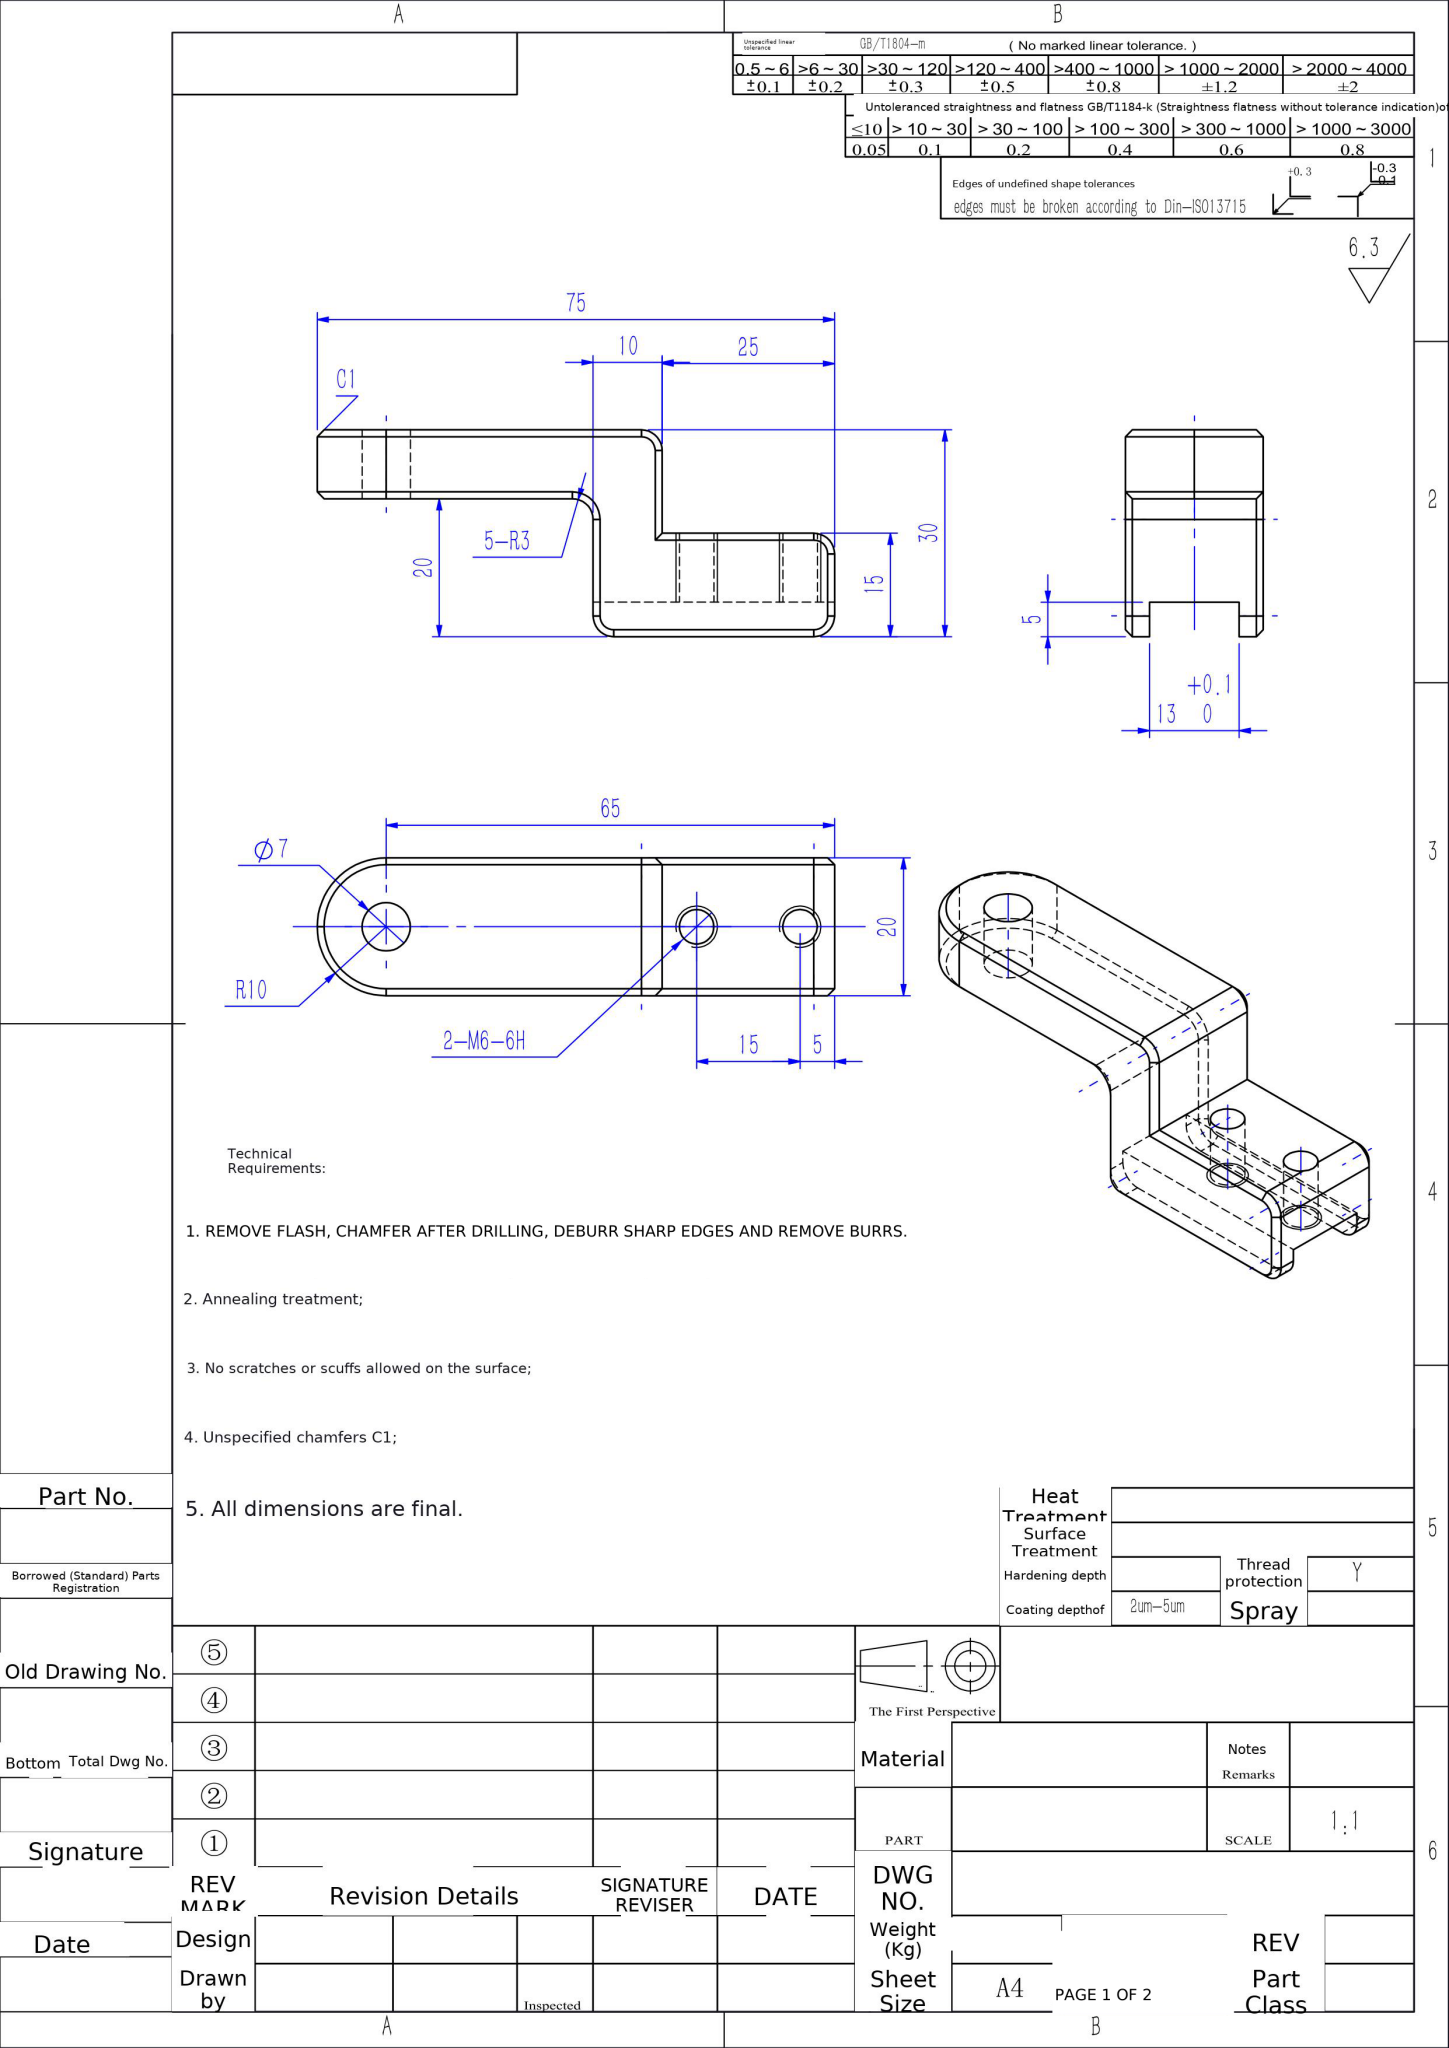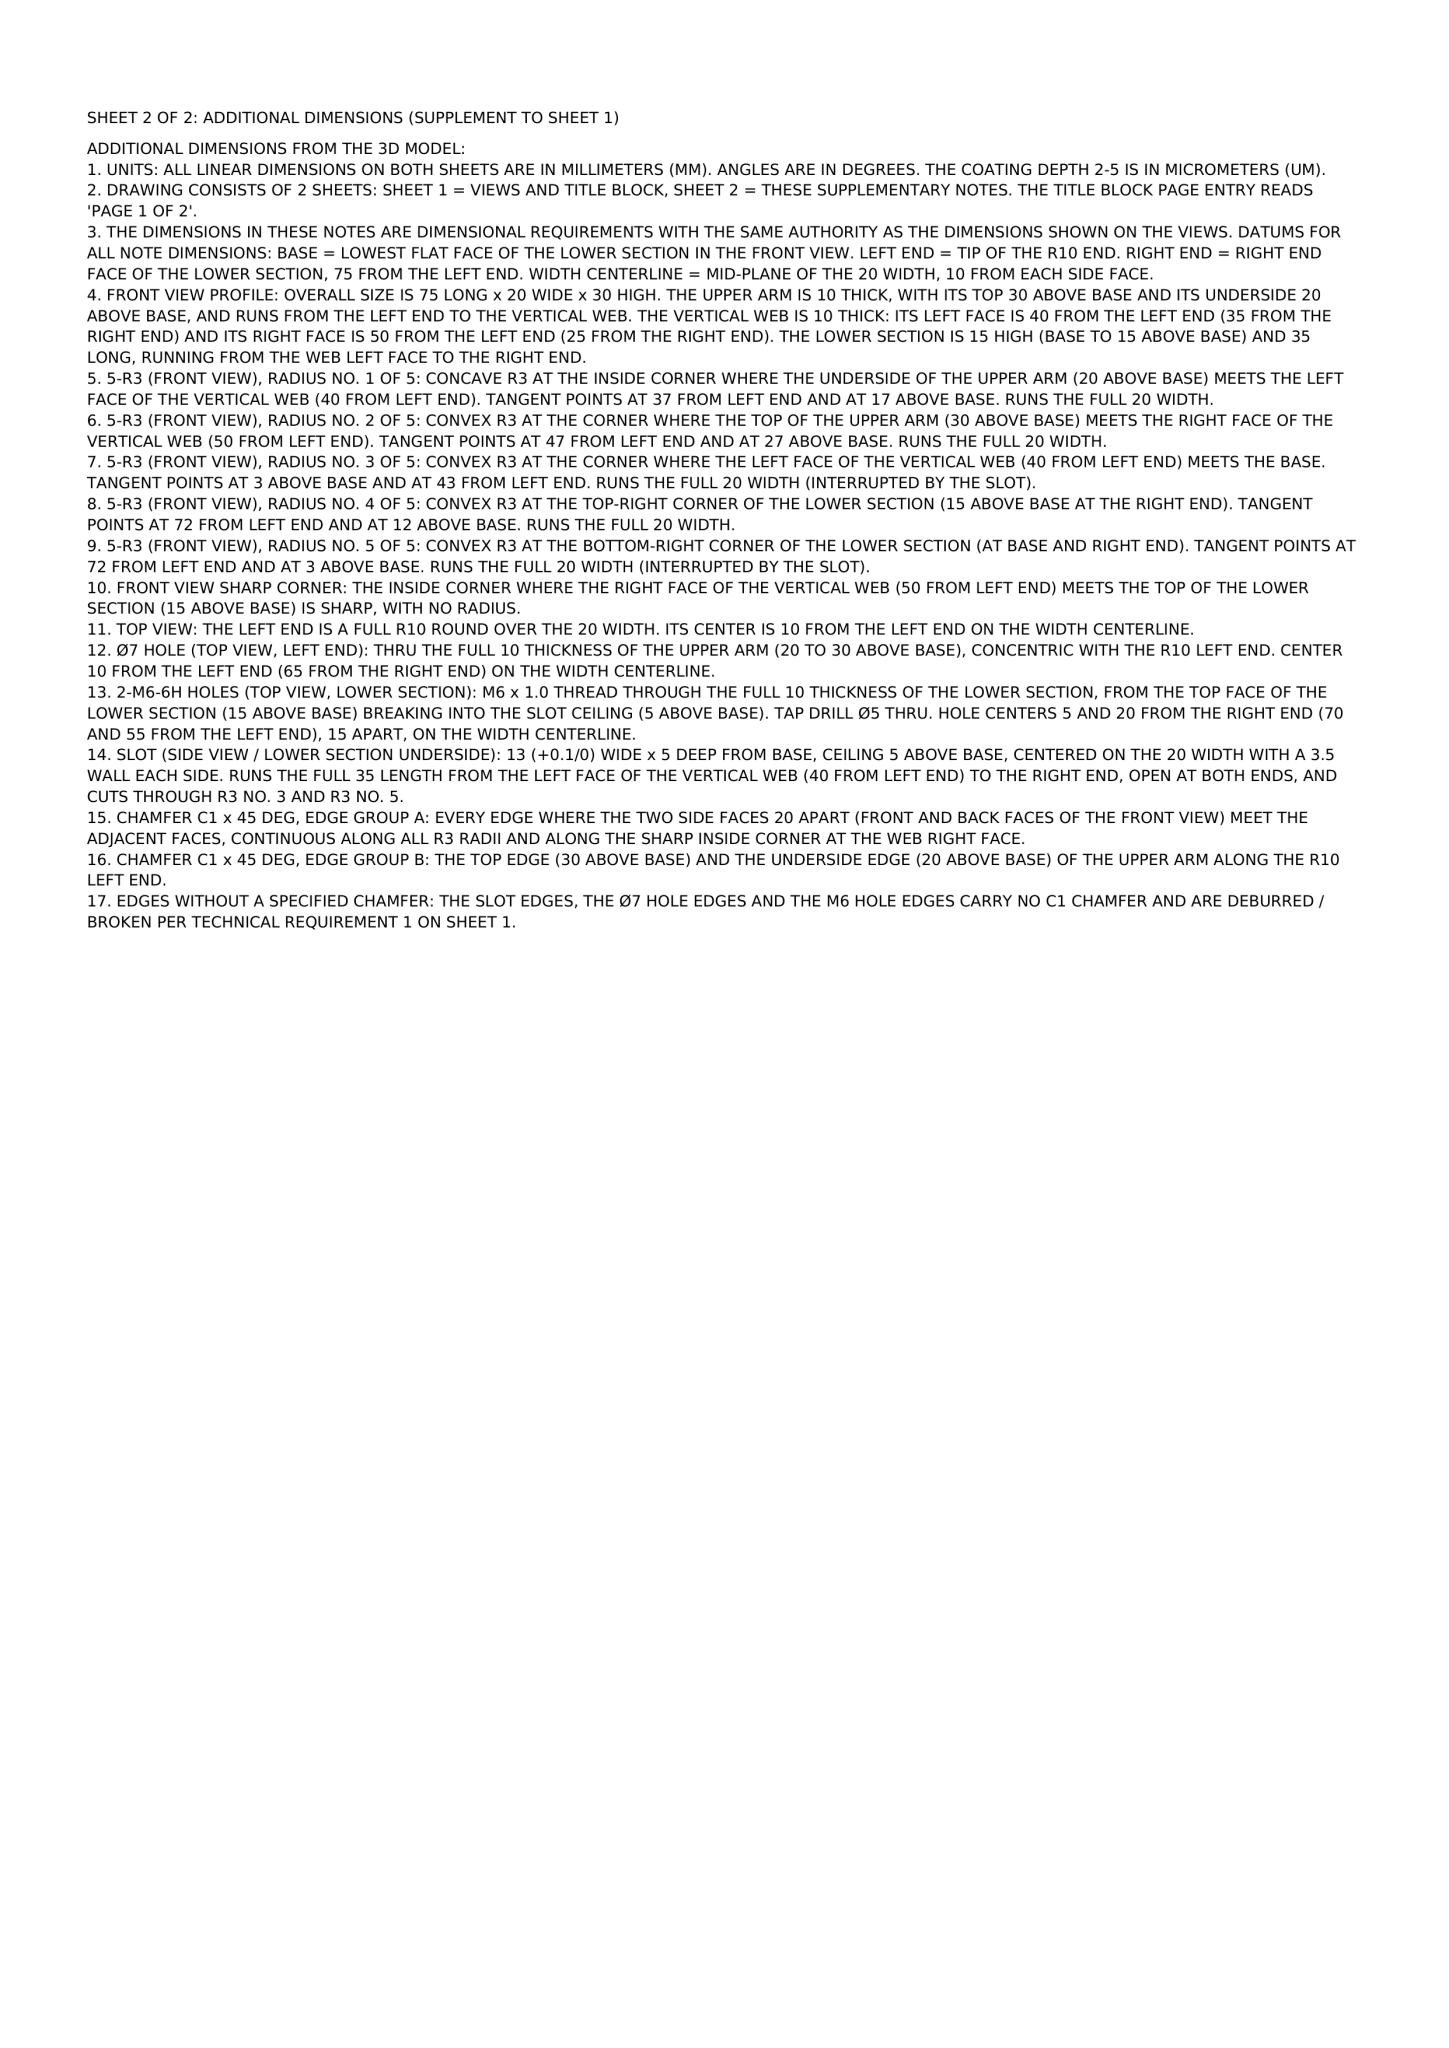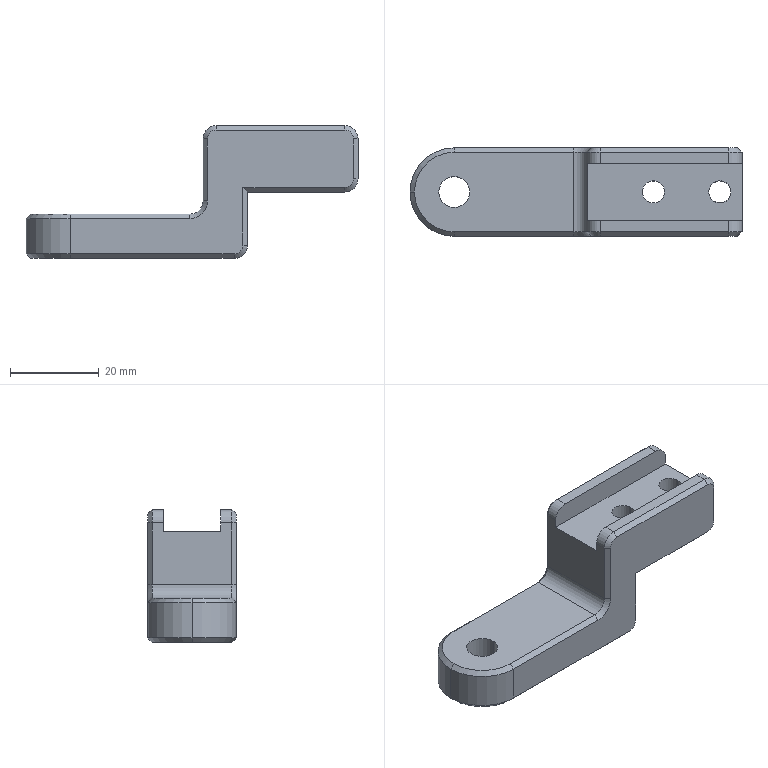Part | NX | mm | 1 solid | 56 faces | box 75 x 20 x 30 mm | volume 17750 mm3 | plane 27 | cylinder 15 | cone 14 | commonest cylinder face diameters 6 x7 5 x4 7 x2 20 x2